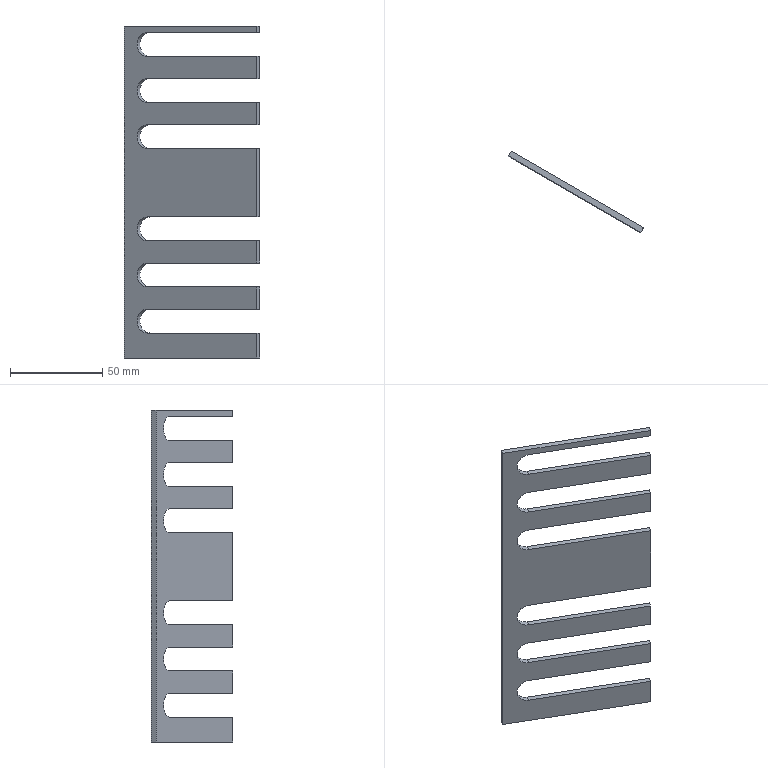Component | SolidWorks | KLHFH017AdjustmentShim-1 | 1 solid | 30 faces | box 73.38 x 44.1 x 180 mm | volume 27596 mm3 | plane 24 | cylinder 6 | commonest cylinder face diameters 13 x6 | material Plain Carbon Steel
STEP:
#1=COLOUR_RGB('',0.7922,0.8196,0.9333);
#2=FILL_AREA_STYLE_COLOUR('',#1);
#3=FILL_AREA_STYLE('',(#2));
#4=SURFACE_STYLE_FILL_AREA(#3);
#5=SURFACE_SIDE_STYLE('',(#4));
#6=SURFACE_STYLE_USAGE(.BOTH.,#5);
#7=PRESENTATION_STYLE_ASSIGNMENT((#6));
#8=CARTESIAN_POINT('',(6.04,7.196,-8.11));
#9=VERTEX_POINT('',#8);
#10=CARTESIAN_POINT('',(5.981,7.094,-8.11));
#11=VERTEX_POINT('',#10);
#12=CARTESIAN_POINT('',(6.04,7.196,-8.11));
#13=DIRECTION('',(-0.5,-0.866,0.));
#14=VECTOR('',#13,39.37);
#15=LINE('',#12,#14);
#16=EDGE_CURVE('',#9,#11,#15,.T.);
#17=ORIENTED_EDGE('',*,*,#16,.F.);
#18=CARTESIAN_POINT('',(6.04,7.196,-7.638));
#19=VERTEX_POINT('',#18);
#20=CARTESIAN_POINT('',(6.04,7.196,-14.075));
#21=DIRECTION('',(0.,0.,1.));
#22=VECTOR('',#21,39.37);
#23=LINE('',#20,#22);
#24=EDGE_CURVE('',#9,#19,#23,.T.);
#25=ORIENTED_EDGE('',*,*,#24,.T.);
#26=CARTESIAN_POINT('',(5.981,7.094,-7.638));
#27=VERTEX_POINT('',#26);
#28=CARTESIAN_POINT('',(6.04,7.196,-7.638));
#29=DIRECTION('',(-0.5,-0.866,0.));
#30=VECTOR('',#29,39.37);
#31=LINE('',#28,#30);
#32=EDGE_CURVE('',#19,#27,#31,.T.);
#33=ORIENTED_EDGE('',*,*,#32,.T.);
#34=CARTESIAN_POINT('',(5.981,7.094,-14.075));
#35=DIRECTION('',(0.,0.,1.));
#36=VECTOR('',#35,39.37);
#37=LINE('',#34,#36);
#38=EDGE_CURVE('',#11,#27,#37,.T.);
#39=ORIENTED_EDGE('',*,*,#38,.F.);
#40=EDGE_LOOP('',(#17,#25,#33,#39));
#41=FACE_OUTER_BOUND('',#40,.T.);
#42=CARTESIAN_POINT('',(5.981,7.094,-14.075));
#43=DIRECTION('',(0.866,-0.5,0.));
#44=DIRECTION('',(0.,0.,1.));
#45=AXIS2_PLACEMENT_3D('',#42,#43,#44);
#46=PLANE('',#45);
#47=ADVANCED_FACE('',(#41),#46,.T.);
#48=CARTESIAN_POINT('',(6.04,7.196,-13.031));
#49=VERTEX_POINT('',#48);
#50=CARTESIAN_POINT('',(3.704,8.545,-13.031));
#51=VERTEX_POINT('',#50);
#52=CARTESIAN_POINT('',(3.704,8.545,-13.031));
#53=DIRECTION('',(-0.866,0.5,0.));
#54=VECTOR('',#53,39.37);
#55=LINE('',#52,#54);
#56=EDGE_CURVE('',#49,#51,#55,.T.);
#57=ORIENTED_EDGE('',*,*,#56,.T.);
#58=CARTESIAN_POINT('',(3.704,8.545,-13.543));
#59=VERTEX_POINT('',#58);
#60=CARTESIAN_POINT('',(3.704,8.545,-13.287));
#61=DIRECTION('',(-0.5,-0.866,0.));
#62=DIRECTION('',(0.,0.,-1.));
#63=AXIS2_PLACEMENT_3D('',#60,#61,#62);
#64=CIRCLE('',#63,0.2559);
#65=EDGE_CURVE('',#51,#59,#64,.T.);
#66=ORIENTED_EDGE('',*,*,#65,.T.);
#67=CARTESIAN_POINT('',(6.04,7.196,-13.543));
#68=VERTEX_POINT('',#67);
#69=CARTESIAN_POINT('',(3.704,8.545,-13.543));
#70=DIRECTION('',(0.866,-0.5,0.));
#71=VECTOR('',#70,39.37);
#72=LINE('',#69,#71);
#73=EDGE_CURVE('',#59,#68,#72,.T.);
#74=ORIENTED_EDGE('',*,*,#73,.T.);
#75=CARTESIAN_POINT('',(6.04,7.196,-14.075));
#76=VERTEX_POINT('',#75);
#77=CARTESIAN_POINT('',(6.04,7.196,-14.075));
#78=DIRECTION('',(0.,0.,1.));
#79=VECTOR('',#78,39.37);
#80=LINE('',#77,#79);
#81=EDGE_CURVE('',#76,#68,#80,.T.);
#82=ORIENTED_EDGE('',*,*,#81,.F.);
#83=CARTESIAN_POINT('',(3.21,8.83,-14.075));
#84=VERTEX_POINT('',#83);
#85=CARTESIAN_POINT('',(3.21,8.83,-14.075));
#86=DIRECTION('',(-0.866,0.5,0.));
#87=VECTOR('',#86,39.37);
#88=LINE('',#85,#87);
#89=EDGE_CURVE('',#76,#84,#88,.T.);
#90=ORIENTED_EDGE('',*,*,#89,.T.);
#91=CARTESIAN_POINT('',(3.21,8.83,-6.988));
#92=VERTEX_POINT('',#91);
#93=CARTESIAN_POINT('',(3.21,8.83,-14.075));
#94=DIRECTION('',(0.,0.,1.));
#95=VECTOR('',#94,39.37);
#96=LINE('',#93,#95);
#97=EDGE_CURVE('',#84,#92,#96,.T.);
#98=ORIENTED_EDGE('',*,*,#97,.T.);
#99=CARTESIAN_POINT('',(6.04,7.196,-6.988));
#100=VERTEX_POINT('',#99);
#101=CARTESIAN_POINT('',(3.21,8.83,-6.988));
#102=DIRECTION('',(-0.866,0.5,0.));
#103=VECTOR('',#102,39.37);
#104=LINE('',#101,#103);
#105=EDGE_CURVE('',#100,#92,#104,.T.);
#106=ORIENTED_EDGE('',*,*,#105,.F.);
#107=CARTESIAN_POINT('',(6.04,7.196,-7.126));
#108=VERTEX_POINT('',#107);
#109=CARTESIAN_POINT('',(6.04,7.196,-14.075));
#110=DIRECTION('',(0.,0.,1.));
#111=VECTOR('',#110,39.37);
#112=LINE('',#109,#111);
#113=EDGE_CURVE('',#108,#100,#112,.T.);
#114=ORIENTED_EDGE('',*,*,#113,.F.);
#115=CARTESIAN_POINT('',(3.704,8.545,-7.126));
#116=VERTEX_POINT('',#115);
#117=CARTESIAN_POINT('',(3.704,8.545,-7.126));
#118=DIRECTION('',(-0.866,0.5,-0.));
#119=VECTOR('',#118,39.37);
#120=LINE('',#117,#119);
#121=EDGE_CURVE('',#108,#116,#120,.T.);
#122=ORIENTED_EDGE('',*,*,#121,.T.);
#123=CARTESIAN_POINT('',(3.704,8.545,-7.638));
#124=VERTEX_POINT('',#123);
#125=CARTESIAN_POINT('',(3.704,8.545,-7.382));
#126=DIRECTION('',(-0.5,-0.866,0.));
#127=DIRECTION('',(0.,0.,-1.));
#128=AXIS2_PLACEMENT_3D('',#125,#126,#127);
#129=CIRCLE('',#128,0.2559);
#130=EDGE_CURVE('',#116,#124,#129,.T.);
#131=ORIENTED_EDGE('',*,*,#130,.T.);
#132=CARTESIAN_POINT('',(3.704,8.545,-7.638));
#133=DIRECTION('',(0.866,-0.5,-0.));
#134=VECTOR('',#133,39.37);
#135=LINE('',#132,#134);
#136=EDGE_CURVE('',#124,#19,#135,.T.);
#137=ORIENTED_EDGE('',*,*,#136,.T.);
#138=ORIENTED_EDGE('',*,*,#24,.F.);
#139=CARTESIAN_POINT('',(3.704,8.545,-8.11));
#140=VERTEX_POINT('',#139);
#141=CARTESIAN_POINT('',(3.704,8.545,-8.11));
#142=DIRECTION('',(-0.866,0.5,0.));
#143=VECTOR('',#142,39.37);
#144=LINE('',#141,#143);
#145=EDGE_CURVE('',#9,#140,#144,.T.);
#146=ORIENTED_EDGE('',*,*,#145,.T.);
#147=CARTESIAN_POINT('',(3.704,8.545,-8.622));
#148=VERTEX_POINT('',#147);
#149=CARTESIAN_POINT('',(3.704,8.545,-8.366));
#150=DIRECTION('',(-0.5,-0.866,0.));
#151=DIRECTION('',(0.,0.,-1.));
#152=AXIS2_PLACEMENT_3D('',#149,#150,#151);
#153=CIRCLE('',#152,0.2559);
#154=EDGE_CURVE('',#140,#148,#153,.T.);
#155=ORIENTED_EDGE('',*,*,#154,.T.);
#156=CARTESIAN_POINT('',(6.04,7.196,-8.622));
#157=VERTEX_POINT('',#156);
#158=CARTESIAN_POINT('',(3.704,8.545,-8.622));
#159=DIRECTION('',(0.866,-0.5,0.));
#160=VECTOR('',#159,39.37);
#161=LINE('',#158,#160);
#162=EDGE_CURVE('',#148,#157,#161,.T.);
#163=ORIENTED_EDGE('',*,*,#162,.T.);
#164=CARTESIAN_POINT('',(6.04,7.196,-9.094));
#165=VERTEX_POINT('',#164);
#166=CARTESIAN_POINT('',(6.04,7.196,-14.075));
#167=DIRECTION('',(0.,0.,1.));
#168=VECTOR('',#167,39.37);
#169=LINE('',#166,#168);
#170=EDGE_CURVE('',#165,#157,#169,.T.);
#171=ORIENTED_EDGE('',*,*,#170,.F.);
#172=CARTESIAN_POINT('',(3.704,8.545,-9.094));
#173=VERTEX_POINT('',#172);
#174=CARTESIAN_POINT('',(3.704,8.545,-9.094));
#175=DIRECTION('',(-0.866,0.5,0.));
#176=VECTOR('',#175,39.37);
#177=LINE('',#174,#176);
#178=EDGE_CURVE('',#165,#173,#177,.T.);
#179=ORIENTED_EDGE('',*,*,#178,.T.);
#180=CARTESIAN_POINT('',(3.704,8.545,-9.606));
#181=VERTEX_POINT('',#180);
#182=CARTESIAN_POINT('',(3.704,8.545,-9.35));
#183=DIRECTION('',(-0.5,-0.866,0.));
#184=DIRECTION('',(0.,0.,-1.));
#185=AXIS2_PLACEMENT_3D('',#182,#183,#184);
#186=CIRCLE('',#185,0.2559);
#187=EDGE_CURVE('',#173,#181,#186,.T.);
#188=ORIENTED_EDGE('',*,*,#187,.T.);
#189=CARTESIAN_POINT('',(6.04,7.196,-9.606));
#190=VERTEX_POINT('',#189);
#191=CARTESIAN_POINT('',(3.704,8.545,-9.606));
#192=DIRECTION('',(0.866,-0.5,0.));
#193=VECTOR('',#192,39.37);
#194=LINE('',#191,#193);
#195=EDGE_CURVE('',#181,#190,#194,.T.);
#196=ORIENTED_EDGE('',*,*,#195,.T.);
#197=CARTESIAN_POINT('',(6.04,7.196,-11.063));
#198=VERTEX_POINT('',#197);
#199=CARTESIAN_POINT('',(6.04,7.196,-14.075));
#200=DIRECTION('',(0.,0.,1.));
#201=VECTOR('',#200,39.37);
#202=LINE('',#199,#201);
#203=EDGE_CURVE('',#198,#190,#202,.T.);
#204=ORIENTED_EDGE('',*,*,#203,.F.);
#205=CARTESIAN_POINT('',(3.704,8.545,-11.063));
#206=VERTEX_POINT('',#205);
#207=CARTESIAN_POINT('',(3.704,8.545,-11.063));
#208=DIRECTION('',(-0.866,0.5,0.));
#209=VECTOR('',#208,39.37);
#210=LINE('',#207,#209);
#211=EDGE_CURVE('',#198,#206,#210,.T.);
#212=ORIENTED_EDGE('',*,*,#211,.T.);
#213=CARTESIAN_POINT('',(3.704,8.545,-11.575));
#214=VERTEX_POINT('',#213);
#215=CARTESIAN_POINT('',(3.704,8.545,-11.319));
#216=DIRECTION('',(-0.5,-0.866,0.));
#217=DIRECTION('',(0.,0.,-1.));
#218=AXIS2_PLACEMENT_3D('',#215,#216,#217);
#219=CIRCLE('',#218,0.2559);
#220=EDGE_CURVE('',#206,#214,#219,.T.);
#221=ORIENTED_EDGE('',*,*,#220,.T.);
#222=CARTESIAN_POINT('',(6.04,7.196,-11.575));
#223=VERTEX_POINT('',#222);
#224=CARTESIAN_POINT('',(3.704,8.545,-11.575));
#225=DIRECTION('',(0.866,-0.5,0.));
#226=VECTOR('',#225,39.37);
#227=LINE('',#224,#226);
#228=EDGE_CURVE('',#214,#223,#227,.T.);
#229=ORIENTED_EDGE('',*,*,#228,.T.);
#230=CARTESIAN_POINT('',(6.04,7.196,-12.047));
#231=VERTEX_POINT('',#230);
#232=CARTESIAN_POINT('',(6.04,7.196,-14.075));
#233=DIRECTION('',(0.,0.,1.));
#234=VECTOR('',#233,39.37);
#235=LINE('',#232,#234);
#236=EDGE_CURVE('',#231,#223,#235,.T.);
#237=ORIENTED_EDGE('',*,*,#236,.F.);
#238=CARTESIAN_POINT('',(3.704,8.545,-12.047));
#239=VERTEX_POINT('',#238);
#240=CARTESIAN_POINT('',(3.704,8.545,-12.047));
#241=DIRECTION('',(-0.866,0.5,0.));
#242=VECTOR('',#241,39.37);
#243=LINE('',#240,#242);
#244=EDGE_CURVE('',#231,#239,#243,.T.);
#245=ORIENTED_EDGE('',*,*,#244,.T.);
#246=CARTESIAN_POINT('',(3.704,8.545,-12.559));
#247=VERTEX_POINT('',#246);
#248=CARTESIAN_POINT('',(3.704,8.545,-12.303));
#249=DIRECTION('',(-0.5,-0.866,0.));
#250=DIRECTION('',(0.,0.,-1.));
#251=AXIS2_PLACEMENT_3D('',#248,#249,#250);
#252=CIRCLE('',#251,0.2559);
#253=EDGE_CURVE('',#239,#247,#252,.T.);
#254=ORIENTED_EDGE('',*,*,#253,.T.);
#255=CARTESIAN_POINT('',(6.04,7.196,-12.559));
#256=VERTEX_POINT('',#255);
#257=CARTESIAN_POINT('',(3.704,8.545,-12.559));
#258=DIRECTION('',(0.866,-0.5,0.));
#259=VECTOR('',#258,39.37);
#260=LINE('',#257,#259);
#261=EDGE_CURVE('',#247,#256,#260,.T.);
#262=ORIENTED_EDGE('',*,*,#261,.T.);
#263=CARTESIAN_POINT('',(6.04,7.196,-14.075));
#264=DIRECTION('',(0.,0.,1.));
#265=VECTOR('',#264,39.37);
#266=LINE('',#263,#265);
#267=EDGE_CURVE('',#49,#256,#266,.T.);
#268=ORIENTED_EDGE('',*,*,#267,.F.);
#269=EDGE_LOOP('',(#57,#66,#74,#82,#90,#98,#106,#114,#122,#131,#137,#138,#146,#155,#163,#171,#179,#188,#196,#204,#212,#221,#229,#237,#245,#254,#262,#268));
#270=FACE_OUTER_BOUND('',#269,.T.);
#271=CARTESIAN_POINT('',(3.21,8.83,-14.075));
#272=DIRECTION('',(0.5,0.866,-0.));
#273=DIRECTION('',(0.,0.,1.));
#274=AXIS2_PLACEMENT_3D('',#271,#272,#273);
#275=PLANE('',#274);
#276=ADVANCED_FACE('',(#270),#275,.T.);
#277=CARTESIAN_POINT('',(5.981,7.094,-12.047));
#278=VERTEX_POINT('',#277);
#279=CARTESIAN_POINT('',(6.04,7.196,-12.047));
#280=DIRECTION('',(-0.5,-0.866,0.));
#281=VECTOR('',#280,39.37);
#282=LINE('',#279,#281);
#283=EDGE_CURVE('',#231,#278,#282,.T.);
#284=ORIENTED_EDGE('',*,*,#283,.F.);
#285=ORIENTED_EDGE('',*,*,#236,.T.);
#286=CARTESIAN_POINT('',(5.981,7.094,-11.575));
#287=VERTEX_POINT('',#286);
#288=CARTESIAN_POINT('',(6.04,7.196,-11.575));
#289=DIRECTION('',(-0.5,-0.866,0.));
#290=VECTOR('',#289,39.37);
#291=LINE('',#288,#290);
#292=EDGE_CURVE('',#223,#287,#291,.T.);
#293=ORIENTED_EDGE('',*,*,#292,.T.);
#294=CARTESIAN_POINT('',(5.981,7.094,-14.075));
#295=DIRECTION('',(0.,0.,1.));
#296=VECTOR('',#295,39.37);
#297=LINE('',#294,#296);
#298=EDGE_CURVE('',#278,#287,#297,.T.);
#299=ORIENTED_EDGE('',*,*,#298,.F.);
#300=EDGE_LOOP('',(#284,#285,#293,#299));
#301=FACE_OUTER_BOUND('',#300,.T.);
#302=CARTESIAN_POINT('',(5.981,7.094,-14.075));
#303=DIRECTION('',(0.866,-0.5,0.));
#304=DIRECTION('',(0.,0.,1.));
#305=AXIS2_PLACEMENT_3D('',#302,#303,#304);
#306=PLANE('',#305);
#307=ADVANCED_FACE('',(#301),#306,.T.);
#308=CARTESIAN_POINT('',(3.645,8.442,-13.031));
#309=VERTEX_POINT('',#308);
#310=CARTESIAN_POINT('',(3.645,8.442,-13.543));
#311=VERTEX_POINT('',#310);
#312=CARTESIAN_POINT('',(3.645,8.442,-13.287));
#313=DIRECTION('',(-0.5,-0.866,0.));
#314=DIRECTION('',(0.,0.,-1.));
#315=AXIS2_PLACEMENT_3D('',#312,#313,#314);
#316=CIRCLE('',#315,0.2559);
#317=EDGE_CURVE('',#309,#311,#316,.T.);
#318=ORIENTED_EDGE('',*,*,#317,.F.);
#319=CARTESIAN_POINT('',(5.981,7.094,-13.031));
#320=VERTEX_POINT('',#319);
#321=CARTESIAN_POINT('',(3.645,8.442,-13.031));
#322=DIRECTION('',(-0.866,0.5,0.));
#323=VECTOR('',#322,39.37);
#324=LINE('',#321,#323);
#325=EDGE_CURVE('',#320,#309,#324,.T.);
#326=ORIENTED_EDGE('',*,*,#325,.F.);
#327=CARTESIAN_POINT('',(5.981,7.094,-12.559));
#328=VERTEX_POINT('',#327);
#329=CARTESIAN_POINT('',(5.981,7.094,-14.075));
#330=DIRECTION('',(0.,0.,1.));
#331=VECTOR('',#330,39.37);
#332=LINE('',#329,#331);
#333=EDGE_CURVE('',#320,#328,#332,.T.);
#334=ORIENTED_EDGE('',*,*,#333,.T.);
#335=CARTESIAN_POINT('',(3.645,8.442,-12.559));
#336=VERTEX_POINT('',#335);
#337=CARTESIAN_POINT('',(3.645,8.442,-12.559));
#338=DIRECTION('',(0.866,-0.5,0.));
#339=VECTOR('',#338,39.37);
#340=LINE('',#337,#339);
#341=EDGE_CURVE('',#336,#328,#340,.T.);
#342=ORIENTED_EDGE('',*,*,#341,.F.);
#343=CARTESIAN_POINT('',(3.645,8.442,-12.047));
#344=VERTEX_POINT('',#343);
#345=CARTESIAN_POINT('',(3.645,8.442,-12.303));
#346=DIRECTION('',(-0.5,-0.866,0.));
#347=DIRECTION('',(0.,0.,-1.));
#348=AXIS2_PLACEMENT_3D('',#345,#346,#347);
#349=CIRCLE('',#348,0.2559);
#350=EDGE_CURVE('',#344,#336,#349,.T.);
#351=ORIENTED_EDGE('',*,*,#350,.F.);
#352=CARTESIAN_POINT('',(3.645,8.442,-12.047));
#353=DIRECTION('',(-0.866,0.5,0.));
#354=VECTOR('',#353,39.37);
#355=LINE('',#352,#354);
#356=EDGE_CURVE('',#278,#344,#355,.T.);
#357=ORIENTED_EDGE('',*,*,#356,.F.);
#358=ORIENTED_EDGE('',*,*,#298,.T.);
#359=CARTESIAN_POINT('',(3.645,8.442,-11.575));
#360=VERTEX_POINT('',#359);
#361=CARTESIAN_POINT('',(3.645,8.442,-11.575));
#362=DIRECTION('',(0.866,-0.5,0.));
#363=VECTOR('',#362,39.37);
#364=LINE('',#361,#363);
#365=EDGE_CURVE('',#360,#287,#364,.T.);
#366=ORIENTED_EDGE('',*,*,#365,.F.);
#367=CARTESIAN_POINT('',(3.645,8.442,-11.063));
#368=VERTEX_POINT('',#367);
#369=CARTESIAN_POINT('',(3.645,8.442,-11.319));
#370=DIRECTION('',(-0.5,-0.866,0.));
#371=DIRECTION('',(0.,0.,-1.));
#372=AXIS2_PLACEMENT_3D('',#369,#370,#371);
#373=CIRCLE('',#372,0.2559);
#374=EDGE_CURVE('',#368,#360,#373,.T.);
#375=ORIENTED_EDGE('',*,*,#374,.F.);
#376=CARTESIAN_POINT('',(5.981,7.094,-11.063));
#377=VERTEX_POINT('',#376);
#378=CARTESIAN_POINT('',(3.645,8.442,-11.063));
#379=DIRECTION('',(-0.866,0.5,0.));
#380=VECTOR('',#379,39.37);
#381=LINE('',#378,#380);
#382=EDGE_CURVE('',#377,#368,#381,.T.);
#383=ORIENTED_EDGE('',*,*,#382,.F.);
#384=CARTESIAN_POINT('',(5.981,7.094,-9.606));
#385=VERTEX_POINT('',#384);
#386=CARTESIAN_POINT('',(5.981,7.094,-14.075));
#387=DIRECTION('',(0.,0.,1.));
#388=VECTOR('',#387,39.37);
#389=LINE('',#386,#388);
#390=EDGE_CURVE('',#377,#385,#389,.T.);
#391=ORIENTED_EDGE('',*,*,#390,.T.);
#392=CARTESIAN_POINT('',(3.645,8.442,-9.606));
#393=VERTEX_POINT('',#392);
#394=CARTESIAN_POINT('',(3.645,8.442,-9.606));
#395=DIRECTION('',(0.866,-0.5,0.));
#396=VECTOR('',#395,39.37);
#397=LINE('',#394,#396);
#398=EDGE_CURVE('',#393,#385,#397,.T.);
#399=ORIENTED_EDGE('',*,*,#398,.F.);
#400=CARTESIAN_POINT('',(3.645,8.442,-9.094));
#401=VERTEX_POINT('',#400);
#402=CARTESIAN_POINT('',(3.645,8.442,-9.35));
#403=DIRECTION('',(-0.5,-0.866,0.));
#404=DIRECTION('',(0.,0.,-1.));
#405=AXIS2_PLACEMENT_3D('',#402,#403,#404);
#406=CIRCLE('',#405,0.2559);
#407=EDGE_CURVE('',#401,#393,#406,.T.);
#408=ORIENTED_EDGE('',*,*,#407,.F.);
#409=CARTESIAN_POINT('',(5.981,7.094,-9.094));
#410=VERTEX_POINT('',#409);
#411=CARTESIAN_POINT('',(3.645,8.442,-9.094));
#412=DIRECTION('',(-0.866,0.5,0.));
#413=VECTOR('',#412,39.37);
#414=LINE('',#411,#413);
#415=EDGE_CURVE('',#410,#401,#414,.T.);
#416=ORIENTED_EDGE('',*,*,#415,.F.);
#417=CARTESIAN_POINT('',(5.981,7.094,-8.622));
#418=VERTEX_POINT('',#417);
#419=CARTESIAN_POINT('',(5.981,7.094,-14.075));
#420=DIRECTION('',(0.,0.,1.));
#421=VECTOR('',#420,39.37);
#422=LINE('',#419,#421);
#423=EDGE_CURVE('',#410,#418,#422,.T.);
#424=ORIENTED_EDGE('',*,*,#423,.T.);
#425=CARTESIAN_POINT('',(3.645,8.442,-8.622));
#426=VERTEX_POINT('',#425);
#427=CARTESIAN_POINT('',(3.645,8.442,-8.622));
#428=DIRECTION('',(0.866,-0.5,0.));
#429=VECTOR('',#428,39.37);
#430=LINE('',#427,#429);
#431=EDGE_CURVE('',#426,#418,#430,.T.);
#432=ORIENTED_EDGE('',*,*,#431,.F.);
#433=CARTESIAN_POINT('',(3.645,8.442,-8.11));
#434=VERTEX_POINT('',#433);
#435=CARTESIAN_POINT('',(3.645,8.442,-8.366));
#436=DIRECTION('',(-0.5,-0.866,0.));
#437=DIRECTION('',(0.,0.,-1.));
#438=AXIS2_PLACEMENT_3D('',#435,#436,#437);
#439=CIRCLE('',#438,0.2559);
#440=EDGE_CURVE('',#434,#426,#439,.T.);
#441=ORIENTED_EDGE('',*,*,#440,.F.);
#442=CARTESIAN_POINT('',(3.645,8.442,-8.11));
#443=DIRECTION('',(-0.866,0.5,0.));
#444=VECTOR('',#443,39.37);
#445=LINE('',#442,#444);
#446=EDGE_CURVE('',#11,#434,#445,.T.);
#447=ORIENTED_EDGE('',*,*,#446,.F.);
#448=ORIENTED_EDGE('',*,*,#38,.T.);
#449=CARTESIAN_POINT('',(3.645,8.442,-7.638));
#450=VERTEX_POINT('',#449);
#451=CARTESIAN_POINT('',(3.645,8.442,-7.638));
#452=DIRECTION('',(0.866,-0.5,-0.));
#453=VECTOR('',#452,39.37);
#454=LINE('',#451,#453);
#455=EDGE_CURVE('',#450,#27,#454,.T.);
#456=ORIENTED_EDGE('',*,*,#455,.F.);
#457=CARTESIAN_POINT('',(3.645,8.442,-7.126));
#458=VERTEX_POINT('',#457);
#459=CARTESIAN_POINT('',(3.645,8.442,-7.382));
#460=DIRECTION('',(-0.5,-0.866,0.));
#461=DIRECTION('',(0.,0.,-1.));
#462=AXIS2_PLACEMENT_3D('',#459,#460,#461);
#463=CIRCLE('',#462,0.2559);
#464=EDGE_CURVE('',#458,#450,#463,.T.);
#465=ORIENTED_EDGE('',*,*,#464,.F.);
#466=CARTESIAN_POINT('',(5.981,7.094,-7.126));
#467=VERTEX_POINT('',#466);
#468=CARTESIAN_POINT('',(3.645,8.442,-7.126));
#469=DIRECTION('',(-0.866,0.5,-0.));
#470=VECTOR('',#469,39.37);
#471=LINE('',#468,#470);
#472=EDGE_CURVE('',#467,#458,#471,.T.);
#473=ORIENTED_EDGE('',*,*,#472,.F.);
#474=CARTESIAN_POINT('',(5.981,7.094,-6.988));
#475=VERTEX_POINT('',#474);
#476=CARTESIAN_POINT('',(5.981,7.094,-14.075));
#477=DIRECTION('',(0.,0.,1.));
#478=VECTOR('',#477,39.37);
#479=LINE('',#476,#478);
#480=EDGE_CURVE('',#467,#475,#479,.T.);
#481=ORIENTED_EDGE('',*,*,#480,.T.);
#482=CARTESIAN_POINT('',(3.151,8.728,-6.988));
#483=VERTEX_POINT('',#482);
#484=CARTESIAN_POINT('',(3.151,8.728,-6.988));
#485=DIRECTION('',(-0.866,0.5,0.));
#486=VECTOR('',#485,39.37);
#487=LINE('',#484,#486);
#488=EDGE_CURVE('',#475,#483,#487,.T.);
#489=ORIENTED_EDGE('',*,*,#488,.T.);
#490=CARTESIAN_POINT('',(3.151,8.728,-14.075));
#491=VERTEX_POINT('',#490);
#492=CARTESIAN_POINT('',(3.151,8.728,-14.075));
#493=DIRECTION('',(0.,0.,1.));
#494=VECTOR('',#493,39.37);
#495=LINE('',#492,#494);
#496=EDGE_CURVE('',#491,#483,#495,.T.);
#497=ORIENTED_EDGE('',*,*,#496,.F.);
#498=CARTESIAN_POINT('',(5.981,7.094,-14.075));
#499=VERTEX_POINT('',#498);
#500=CARTESIAN_POINT('',(3.151,8.728,-14.075));
#501=DIRECTION('',(-0.866,0.5,0.));
#502=VECTOR('',#501,39.37);
#503=LINE('',#500,#502);
#504=EDGE_CURVE('',#499,#491,#503,.T.);
#505=ORIENTED_EDGE('',*,*,#504,.F.);
#506=CARTESIAN_POINT('',(5.981,7.094,-13.543));
#507=VERTEX_POINT('',#506);
#508=CARTESIAN_POINT('',(5.981,7.094,-14.075));
#509=DIRECTION('',(0.,0.,1.));
#510=VECTOR('',#509,39.37);
#511=LINE('',#508,#510);
#512=EDGE_CURVE('',#499,#507,#511,.T.);
#513=ORIENTED_EDGE('',*,*,#512,.T.);
#514=CARTESIAN_POINT('',(3.645,8.442,-13.543));
#515=DIRECTION('',(0.866,-0.5,0.));
#516=VECTOR('',#515,39.37);
#517=LINE('',#514,#516);
#518=EDGE_CURVE('',#311,#507,#517,.T.);
#519=ORIENTED_EDGE('',*,*,#518,.F.);
#520=EDGE_LOOP('',(#318,#326,#334,#342,#351,#357,#358,#366,#375,#383,#391,#399,#408,#416,#424,#432,#441,#447,#448,#456,#465,#473,#481,#489,#497,#505,#513,#519));
#521=FACE_OUTER_BOUND('',#520,.T.);
#522=CARTESIAN_POINT('',(3.151,8.728,-14.075));
#523=DIRECTION('',(0.5,0.866,-0.));
#524=DIRECTION('',(0.,0.,1.));
#525=AXIS2_PLACEMENT_3D('',#522,#523,#524);
#526=PLANE('',#525);
#527=ADVANCED_FACE('',(#521),#526,.F.);
#528=CARTESIAN_POINT('',(6.04,7.196,-7.126));
#529=DIRECTION('',(-0.5,-0.866,0.));
#530=VECTOR('',#529,39.37);
#531=LINE('',#528,#530);
#532=EDGE_CURVE('',#108,#467,#531,.T.);
#533=ORIENTED_EDGE('',*,*,#532,.F.);
#534=ORIENTED_EDGE('',*,*,#113,.T.);
#535=CARTESIAN_POINT('',(5.981,7.094,-6.988));
#536=DIRECTION('',(0.5,0.866,-0.));
#537=VECTOR('',#536,39.37);
#538=LINE('',#535,#537);
#539=EDGE_CURVE('',#475,#100,#538,.T.);
#540=ORIENTED_EDGE('',*,*,#539,.F.);
#541=ORIENTED_EDGE('',*,*,#480,.F.);
#542=EDGE_LOOP('',(#533,#534,#540,#541));
#543=FACE_OUTER_BOUND('',#542,.T.);
#544=CARTESIAN_POINT('',(5.981,7.094,-14.075));
#545=DIRECTION('',(0.866,-0.5,0.));
#546=DIRECTION('',(0.,0.,1.));
#547=AXIS2_PLACEMENT_3D('',#544,#545,#546);
#548=PLANE('',#547);
#549=ADVANCED_FACE('',(#543),#548,.T.);
#550=CARTESIAN_POINT('',(6.04,7.196,-9.094));
#551=DIRECTION('',(-0.5,-0.866,0.));
#552=VECTOR('',#551,39.37);
#553=LINE('',#550,#552);
#554=EDGE_CURVE('',#165,#410,#553,.T.);
#555=ORIENTED_EDGE('',*,*,#554,.F.);
#556=ORIENTED_EDGE('',*,*,#170,.T.);
#557=CARTESIAN_POINT('',(6.04,7.196,-8.622));
#558=DIRECTION('',(-0.5,-0.866,0.));
#559=VECTOR('',#558,39.37);
#560=LINE('',#557,#559);
#561=EDGE_CURVE('',#157,#418,#560,.T.);
#562=ORIENTED_EDGE('',*,*,#561,.T.);
#563=ORIENTED_EDGE('',*,*,#423,.F.);
#564=EDGE_LOOP('',(#555,#556,#562,#563));
#565=FACE_OUTER_BOUND('',#564,.T.);
#566=CARTESIAN_POINT('',(5.981,7.094,-14.075));
#567=DIRECTION('',(0.866,-0.5,0.));
#568=DIRECTION('',(0.,0.,1.));
#569=AXIS2_PLACEMENT_3D('',#566,#567,#568);
#570=PLANE('',#569);
#571=ADVANCED_FACE('',(#565),#570,.T.);
#572=CARTESIAN_POINT('',(6.04,7.196,-11.063));
#573=DIRECTION('',(-0.5,-0.866,0.));
#574=VECTOR('',#573,39.37);
#575=LINE('',#572,#574);
#576=EDGE_CURVE('',#198,#377,#575,.T.);
#577=ORIENTED_EDGE('',*,*,#576,.F.);
#578=ORIENTED_EDGE('',*,*,#203,.T.);
#579=CARTESIAN_POINT('',(6.04,7.196,-9.606));
#580=DIRECTION('',(-0.5,-0.866,0.));
#581=VECTOR('',#580,39.37);
#582=LINE('',#579,#581);
#583=EDGE_CURVE('',#190,#385,#582,.T.);
#584=ORIENTED_EDGE('',*,*,#583,.T.);
#585=ORIENTED_EDGE('',*,*,#390,.F.);
#586=EDGE_LOOP('',(#577,#578,#584,#585));
#587=FACE_OUTER_BOUND('',#586,.T.);
#588=CARTESIAN_POINT('',(5.981,7.094,-14.075));
#589=DIRECTION('',(0.866,-0.5,0.));
#590=DIRECTION('',(0.,0.,1.));
#591=AXIS2_PLACEMENT_3D('',#588,#589,#590);
#592=PLANE('',#591);
#593=ADVANCED_FACE('',(#587),#592,.T.);
#594=CARTESIAN_POINT('',(6.04,7.196,-13.031));
#595=DIRECTION('',(-0.5,-0.866,0.));
#596=VECTOR('',#595,39.37);
#597=LINE('',#594,#596);
#598=EDGE_CURVE('',#49,#320,#597,.T.);
#599=ORIENTED_EDGE('',*,*,#598,.F.);
#600=ORIENTED_EDGE('',*,*,#267,.T.);
#601=CARTESIAN_POINT('',(6.04,7.196,-12.559));
#602=DIRECTION('',(-0.5,-0.866,0.));
#603=VECTOR('',#602,39.37);
#604=LINE('',#601,#603);
#605=EDGE_CURVE('',#256,#328,#604,.T.);
#606=ORIENTED_EDGE('',*,*,#605,.T.);
#607=ORIENTED_EDGE('',*,*,#333,.F.);
#608=EDGE_LOOP('',(#599,#600,#606,#607));
#609=FACE_OUTER_BOUND('',#608,.T.);
#610=CARTESIAN_POINT('',(5.981,7.094,-14.075));
#611=DIRECTION('',(0.866,-0.5,0.));
#612=DIRECTION('',(0.,0.,1.));
#613=AXIS2_PLACEMENT_3D('',#610,#611,#612);
#614=PLANE('',#613);
#615=ADVANCED_FACE('',(#609),#614,.T.);
#616=CARTESIAN_POINT('',(3.21,8.83,-6.988));
#617=DIRECTION('',(-0.5,-0.866,0.));
#618=VECTOR('',#617,39.37);
#619=LINE('',#616,#618);
#620=EDGE_CURVE('',#92,#483,#619,.T.);
#621=ORIENTED_EDGE('',*,*,#620,.F.);
#622=ORIENTED_EDGE('',*,*,#97,.F.);
#623=CARTESIAN_POINT('',(3.21,8.83,-14.075));
#624=DIRECTION('',(-0.5,-0.866,0.));
#625=VECTOR('',#624,39.37);
#626=LINE('',#623,#625);
#627=EDGE_CURVE('',#84,#491,#626,.T.);
#628=ORIENTED_EDGE('',*,*,#627,.T.);
#629=ORIENTED_EDGE('',*,*,#496,.T.);
#630=EDGE_LOOP('',(#621,#622,#628,#629));
#631=FACE_OUTER_BOUND('',#630,.T.);
#632=CARTESIAN_POINT('',(3.21,8.83,-14.075));
#633=DIRECTION('',(-0.866,0.5,0.));
#634=DIRECTION('',(-0.,-0.,-1.));
#635=AXIS2_PLACEMENT_3D('',#632,#633,#634);
#636=PLANE('',#635);
#637=ADVANCED_FACE('',(#631),#636,.T.);
#638=CARTESIAN_POINT('',(6.04,7.196,-13.543));
#639=DIRECTION('',(-0.5,-0.866,0.));
#640=VECTOR('',#639,39.37);
#641=LINE('',#638,#640);
#642=EDGE_CURVE('',#68,#507,#641,.T.);
#643=ORIENTED_EDGE('',*,*,#642,.T.);
#644=ORIENTED_EDGE('',*,*,#512,.F.);
#645=CARTESIAN_POINT('',(5.981,7.094,-14.075));
#646=DIRECTION('',(0.5,0.866,-0.));
#647=VECTOR('',#646,39.37);
#648=LINE('',#645,#647);
#649=EDGE_CURVE('',#499,#76,#648,.T.);
#650=ORIENTED_EDGE('',*,*,#649,.T.);
#651=ORIENTED_EDGE('',*,*,#81,.T.);
#652=EDGE_LOOP('',(#643,#644,#650,#651));
#653=FACE_OUTER_BOUND('',#652,.T.);
#654=CARTESIAN_POINT('',(5.981,7.094,-14.075));
#655=DIRECTION('',(0.866,-0.5,0.));
#656=DIRECTION('',(0.,0.,1.));
#657=AXIS2_PLACEMENT_3D('',#654,#655,#656);
#658=PLANE('',#657);
#659=ADVANCED_FACE('',(#653),#658,.T.);
#660=ORIENTED_EDGE('',*,*,#504,.T.);
#661=ORIENTED_EDGE('',*,*,#627,.F.);
#662=ORIENTED_EDGE('',*,*,#89,.F.);
#663=ORIENTED_EDGE('',*,*,#649,.F.);
#664=EDGE_LOOP('',(#660,#661,#662,#663));
#665=FACE_OUTER_BOUND('',#664,.T.);
#666=CARTESIAN_POINT('',(3.21,8.83,-14.075));
#667=DIRECTION('',(-0.,-0.,-1.));
#668=DIRECTION('',(0.866,-0.5,0.));
#669=AXIS2_PLACEMENT_3D('',#666,#667,#668);
#670=PLANE('',#669);
#671=ADVANCED_FACE('',(#665),#670,.T.);
#672=ORIENTED_EDGE('',*,*,#488,.F.);
#673=ORIENTED_EDGE('',*,*,#539,.T.);
#674=ORIENTED_EDGE('',*,*,#105,.T.);
#675=ORIENTED_EDGE('',*,*,#620,.T.);
#676=EDGE_LOOP('',(#672,#673,#674,#675));
#677=FACE_OUTER_BOUND('',#676,.T.);
#678=CARTESIAN_POINT('',(3.21,8.83,-6.988));
#679=DIRECTION('',(-0.,-0.,-1.));
#680=DIRECTION('',(0.866,-0.5,0.));
#681=AXIS2_PLACEMENT_3D('',#678,#679,#680);
#682=PLANE('',#681);
#683=ADVANCED_FACE('',(#677),#682,.F.);
#684=ORIENTED_EDGE('',*,*,#464,.T.);
#685=CARTESIAN_POINT('',(3.704,8.545,-7.638));
#686=DIRECTION('',(-0.5,-0.866,0.));
#687=VECTOR('',#686,39.37);
#688=LINE('',#685,#687);
#689=EDGE_CURVE('',#124,#450,#688,.T.);
#690=ORIENTED_EDGE('',*,*,#689,.F.);
#691=ORIENTED_EDGE('',*,*,#130,.F.);
#692=CARTESIAN_POINT('',(3.704,8.545,-7.126));
#693=DIRECTION('',(-0.5,-0.866,0.));
#694=VECTOR('',#693,39.37);
#695=LINE('',#692,#694);
#696=EDGE_CURVE('',#116,#458,#695,.T.);
#697=ORIENTED_EDGE('',*,*,#696,.T.);
#698=EDGE_LOOP('',(#684,#690,#691,#697));
#699=FACE_OUTER_BOUND('',#698,.T.);
#700=CARTESIAN_POINT('',(3.704,8.545,-7.382));
#701=DIRECTION('',(-0.5,-0.866,0.));
#702=DIRECTION('',(0.,0.,-1.));
#703=AXIS2_PLACEMENT_3D('',#700,#701,#702);
#704=CYLINDRICAL_SURFACE('',#703,0.2559);
#705=ADVANCED_FACE('',(#699),#704,.F.);
#706=ORIENTED_EDGE('',*,*,#472,.T.);
#707=ORIENTED_EDGE('',*,*,#696,.F.);
#708=ORIENTED_EDGE('',*,*,#121,.F.);
#709=ORIENTED_EDGE('',*,*,#532,.T.);
#710=EDGE_LOOP('',(#706,#707,#708,#709));
#711=FACE_OUTER_BOUND('',#710,.T.);
#712=CARTESIAN_POINT('',(3.704,8.545,-7.126));
#713=DIRECTION('',(-0.,0.,1.));
#714=DIRECTION('',(-0.866,0.5,-0.));
#715=AXIS2_PLACEMENT_3D('',#712,#713,#714);
#716=PLANE('',#715);
#717=ADVANCED_FACE('',(#711),#716,.F.);
#718=ORIENTED_EDGE('',*,*,#455,.T.);
#719=ORIENTED_EDGE('',*,*,#32,.F.);
#720=ORIENTED_EDGE('',*,*,#136,.F.);
#721=ORIENTED_EDGE('',*,*,#689,.T.);
#722=EDGE_LOOP('',(#718,#719,#720,#721));
#723=FACE_OUTER_BOUND('',#722,.T.);
#724=CARTESIAN_POINT('',(3.704,8.545,-7.638));
#725=DIRECTION('',(-0.,0.,-1.));
#726=DIRECTION('',(0.866,-0.5,-0.));
#727=AXIS2_PLACEMENT_3D('',#724,#725,#726);
#728=PLANE('',#727);
#729=ADVANCED_FACE('',(#723),#728,.F.);
#730=ORIENTED_EDGE('',*,*,#440,.T.);
#731=CARTESIAN_POINT('',(3.704,8.545,-8.622));
#732=DIRECTION('',(-0.5,-0.866,0.));
#733=VECTOR('',#732,39.37);
#734=LINE('',#731,#733);
#735=EDGE_CURVE('',#148,#426,#734,.T.);
#736=ORIENTED_EDGE('',*,*,#735,.F.);
#737=ORIENTED_EDGE('',*,*,#154,.F.);
#738=CARTESIAN_POINT('',(3.704,8.545,-8.11));
#739=DIRECTION('',(-0.5,-0.866,0.));
#740=VECTOR('',#739,39.37);
#741=LINE('',#738,#740);
#742=EDGE_CURVE('',#140,#434,#741,.T.);
#743=ORIENTED_EDGE('',*,*,#742,.T.);
#744=EDGE_LOOP('',(#730,#736,#737,#743));
#745=FACE_OUTER_BOUND('',#744,.T.);
#746=CARTESIAN_POINT('',(3.704,8.545,-8.366));
#747=DIRECTION('',(-0.5,-0.866,0.));
#748=DIRECTION('',(0.,0.,-1.));
#749=AXIS2_PLACEMENT_3D('',#746,#747,#748);
#750=CYLINDRICAL_SURFACE('',#749,0.2559);
#751=ADVANCED_FACE('',(#745),#750,.F.);
#752=ORIENTED_EDGE('',*,*,#446,.T.);
#753=ORIENTED_EDGE('',*,*,#742,.F.);
#754=ORIENTED_EDGE('',*,*,#145,.F.);
#755=ORIENTED_EDGE('',*,*,#16,.T.);
#756=EDGE_LOOP('',(#752,#753,#754,#755));
#757=FACE_OUTER_BOUND('',#756,.T.);
#758=CARTESIAN_POINT('',(3.704,8.545,-8.11));
#759=DIRECTION('',(0.,0.,1.));
#760=DIRECTION('',(-0.866,0.5,0.));
#761=AXIS2_PLACEMENT_3D('',#758,#759,#760);
#762=PLANE('',#761);
#763=ADVANCED_FACE('',(#757),#762,.F.);
#764=ORIENTED_EDGE('',*,*,#431,.T.);
#765=ORIENTED_EDGE('',*,*,#561,.F.);
#766=ORIENTED_EDGE('',*,*,#162,.F.);
#767=ORIENTED_EDGE('',*,*,#735,.T.);
#768=EDGE_LOOP('',(#764,#765,#766,#767));
#769=FACE_OUTER_BOUND('',#768,.T.);
#770=CARTESIAN_POINT('',(3.704,8.545,-8.622));
#771=DIRECTION('',(-0.,-0.,-1.));
#772=DIRECTION('',(0.866,-0.5,0.));
#773=AXIS2_PLACEMENT_3D('',#770,#771,#772);
#774=PLANE('',#773);
#775=ADVANCED_FACE('',(#769),#774,.F.);
#776=ORIENTED_EDGE('',*,*,#407,.T.);
#777=CARTESIAN_POINT('',(3.704,8.545,-9.606));
#778=DIRECTION('',(-0.5,-0.866,0.));
#779=VECTOR('',#778,39.37);
#780=LINE('',#777,#779);
#781=EDGE_CURVE('',#181,#393,#780,.T.);
#782=ORIENTED_EDGE('',*,*,#781,.F.);
#783=ORIENTED_EDGE('',*,*,#187,.F.);
#784=CARTESIAN_POINT('',(3.704,8.545,-9.094));
#785=DIRECTION('',(-0.5,-0.866,0.));
#786=VECTOR('',#785,39.37);
#787=LINE('',#784,#786);
#788=EDGE_CURVE('',#173,#401,#787,.T.);
#789=ORIENTED_EDGE('',*,*,#788,.T.);
#790=EDGE_LOOP('',(#776,#782,#783,#789));
#791=FACE_OUTER_BOUND('',#790,.T.);
#792=CARTESIAN_POINT('',(3.704,8.545,-9.35));
#793=DIRECTION('',(-0.5,-0.866,0.));
#794=DIRECTION('',(0.,0.,-1.));
#795=AXIS2_PLACEMENT_3D('',#792,#793,#794);
#796=CYLINDRICAL_SURFACE('',#795,0.2559);
#797=ADVANCED_FACE('',(#791),#796,.F.);
#798=ORIENTED_EDGE('',*,*,#415,.T.);
#799=ORIENTED_EDGE('',*,*,#788,.F.);
#800=ORIENTED_EDGE('',*,*,#178,.F.);
#801=ORIENTED_EDGE('',*,*,#554,.T.);
#802=EDGE_LOOP('',(#798,#799,#800,#801));
#803=FACE_OUTER_BOUND('',#802,.T.);
#804=CARTESIAN_POINT('',(3.704,8.545,-9.094));
#805=DIRECTION('',(0.,0.,1.));
#806=DIRECTION('',(-0.866,0.5,0.));
#807=AXIS2_PLACEMENT_3D('',#804,#805,#806);
#808=PLANE('',#807);
#809=ADVANCED_FACE('',(#803),#808,.F.);
#810=ORIENTED_EDGE('',*,*,#398,.T.);
#811=ORIENTED_EDGE('',*,*,#583,.F.);
#812=ORIENTED_EDGE('',*,*,#195,.F.);
#813=ORIENTED_EDGE('',*,*,#781,.T.);
#814=EDGE_LOOP('',(#810,#811,#812,#813));
#815=FACE_OUTER_BOUND('',#814,.T.);
#816=CARTESIAN_POINT('',(3.704,8.545,-9.606));
#817=DIRECTION('',(-0.,-0.,-1.));
#818=DIRECTION('',(0.866,-0.5,0.));
#819=AXIS2_PLACEMENT_3D('',#816,#817,#818);
#820=PLANE('',#819);
#821=ADVANCED_FACE('',(#815),#820,.F.);
#822=ORIENTED_EDGE('',*,*,#374,.T.);
#823=CARTESIAN_POINT('',(3.704,8.545,-11.575));
#824=DIRECTION('',(-0.5,-0.866,0.));
#825=VECTOR('',#824,39.37);
#826=LINE('',#823,#825);
#827=EDGE_CURVE('',#214,#360,#826,.T.);
#828=ORIENTED_EDGE('',*,*,#827,.F.);
#829=ORIENTED_EDGE('',*,*,#220,.F.);
#830=CARTESIAN_POINT('',(3.704,8.545,-11.063));
#831=DIRECTION('',(-0.5,-0.866,0.));
#832=VECTOR('',#831,39.37);
#833=LINE('',#830,#832);
#834=EDGE_CURVE('',#206,#368,#833,.T.);
#835=ORIENTED_EDGE('',*,*,#834,.T.);
#836=EDGE_LOOP('',(#822,#828,#829,#835));
#837=FACE_OUTER_BOUND('',#836,.T.);
#838=CARTESIAN_POINT('',(3.704,8.545,-11.319));
#839=DIRECTION('',(-0.5,-0.866,0.));
#840=DIRECTION('',(0.,0.,-1.));
#841=AXIS2_PLACEMENT_3D('',#838,#839,#840);
#842=CYLINDRICAL_SURFACE('',#841,0.2559);
#843=ADVANCED_FACE('',(#837),#842,.F.);
#844=ORIENTED_EDGE('',*,*,#382,.T.);
#845=ORIENTED_EDGE('',*,*,#834,.F.);
#846=ORIENTED_EDGE('',*,*,#211,.F.);
#847=ORIENTED_EDGE('',*,*,#576,.T.);
#848=EDGE_LOOP('',(#844,#845,#846,#847));
#849=FACE_OUTER_BOUND('',#848,.T.);
#850=CARTESIAN_POINT('',(3.704,8.545,-11.063));
#851=DIRECTION('',(0.,0.,1.));
#852=DIRECTION('',(-0.866,0.5,0.));
#853=AXIS2_PLACEMENT_3D('',#850,#851,#852);
#854=PLANE('',#853);
#855=ADVANCED_FACE('',(#849),#854,.F.);
#856=ORIENTED_EDGE('',*,*,#365,.T.);
#857=ORIENTED_EDGE('',*,*,#292,.F.);
#858=ORIENTED_EDGE('',*,*,#228,.F.);
#859=ORIENTED_EDGE('',*,*,#827,.T.);
#860=EDGE_LOOP('',(#856,#857,#858,#859));
#861=FACE_OUTER_BOUND('',#860,.T.);
#862=CARTESIAN_POINT('',(3.704,8.545,-11.575));
#863=DIRECTION('',(-0.,-0.,-1.));
#864=DIRECTION('',(0.866,-0.5,0.));
#865=AXIS2_PLACEMENT_3D('',#862,#863,#864);
#866=PLANE('',#865);
#867=ADVANCED_FACE('',(#861),#866,.F.);
#868=ORIENTED_EDGE('',*,*,#350,.T.);
#869=CARTESIAN_POINT('',(3.704,8.545,-12.559));
#870=DIRECTION('',(-0.5,-0.866,0.));
#871=VECTOR('',#870,39.37);
#872=LINE('',#869,#871);
#873=EDGE_CURVE('',#247,#336,#872,.T.);
#874=ORIENTED_EDGE('',*,*,#873,.F.);
#875=ORIENTED_EDGE('',*,*,#253,.F.);
#876=CARTESIAN_POINT('',(3.704,8.545,-12.047));
#877=DIRECTION('',(-0.5,-0.866,0.));
#878=VECTOR('',#877,39.37);
#879=LINE('',#876,#878);
#880=EDGE_CURVE('',#239,#344,#879,.T.);
#881=ORIENTED_EDGE('',*,*,#880,.T.);
#882=EDGE_LOOP('',(#868,#874,#875,#881));
#883=FACE_OUTER_BOUND('',#882,.T.);
#884=CARTESIAN_POINT('',(3.704,8.545,-12.303));
#885=DIRECTION('',(-0.5,-0.866,0.));
#886=DIRECTION('',(0.,0.,-1.));
#887=AXIS2_PLACEMENT_3D('',#884,#885,#886);
#888=CYLINDRICAL_SURFACE('',#887,0.2559);
#889=ADVANCED_FACE('',(#883),#888,.F.);
#890=ORIENTED_EDGE('',*,*,#356,.T.);
#891=ORIENTED_EDGE('',*,*,#880,.F.);
#892=ORIENTED_EDGE('',*,*,#244,.F.);
#893=ORIENTED_EDGE('',*,*,#283,.T.);
#894=EDGE_LOOP('',(#890,#891,#892,#893));
#895=FACE_OUTER_BOUND('',#894,.T.);
#896=CARTESIAN_POINT('',(3.704,8.545,-12.047));
#897=DIRECTION('',(0.,0.,1.));
#898=DIRECTION('',(-0.866,0.5,0.));
#899=AXIS2_PLACEMENT_3D('',#896,#897,#898);
#900=PLANE('',#899);
#901=ADVANCED_FACE('',(#895),#900,.F.);
#902=ORIENTED_EDGE('',*,*,#341,.T.);
#903=ORIENTED_EDGE('',*,*,#605,.F.);
#904=ORIENTED_EDGE('',*,*,#261,.F.);
#905=ORIENTED_EDGE('',*,*,#873,.T.);
#906=EDGE_LOOP('',(#902,#903,#904,#905));
#907=FACE_OUTER_BOUND('',#906,.T.);
#908=CARTESIAN_POINT('',(3.704,8.545,-12.559));
#909=DIRECTION('',(0.,-0.,-1.));
#910=DIRECTION('',(0.866,-0.5,0.));
#911=AXIS2_PLACEMENT_3D('',#908,#909,#910);
#912=PLANE('',#911);
#913=ADVANCED_FACE('',(#907),#912,.F.);
#914=ORIENTED_EDGE('',*,*,#317,.T.);
#915=CARTESIAN_POINT('',(3.704,8.545,-13.543));
#916=DIRECTION('',(-0.5,-0.866,0.));
#917=VECTOR('',#916,39.37);
#918=LINE('',#915,#917);
#919=EDGE_CURVE('',#59,#311,#918,.T.);
#920=ORIENTED_EDGE('',*,*,#919,.F.);
#921=ORIENTED_EDGE('',*,*,#65,.F.);
#922=CARTESIAN_POINT('',(3.704,8.545,-13.031));
#923=DIRECTION('',(-0.5,-0.866,0.));
#924=VECTOR('',#923,39.37);
#925=LINE('',#922,#924);
#926=EDGE_CURVE('',#51,#309,#925,.T.);
#927=ORIENTED_EDGE('',*,*,#926,.T.);
#928=EDGE_LOOP('',(#914,#920,#921,#927));
#929=FACE_OUTER_BOUND('',#928,.T.);
#930=CARTESIAN_POINT('',(3.704,8.545,-13.287));
#931=DIRECTION('',(-0.5,-0.866,0.));
#932=DIRECTION('',(0.,0.,-1.));
#933=AXIS2_PLACEMENT_3D('',#930,#931,#932);
#934=CYLINDRICAL_SURFACE('',#933,0.2559);
#935=ADVANCED_FACE('',(#929),#934,.F.);
#936=ORIENTED_EDGE('',*,*,#325,.T.);
#937=ORIENTED_EDGE('',*,*,#926,.F.);
#938=ORIENTED_EDGE('',*,*,#56,.F.);
#939=ORIENTED_EDGE('',*,*,#598,.T.);
#940=EDGE_LOOP('',(#936,#937,#938,#939));
#941=FACE_OUTER_BOUND('',#940,.T.);
#942=CARTESIAN_POINT('',(3.704,8.545,-13.031));
#943=DIRECTION('',(0.,0.,1.));
#944=DIRECTION('',(-0.866,0.5,0.));
#945=AXIS2_PLACEMENT_3D('',#942,#943,#944);
#946=PLANE('',#945);
#947=ADVANCED_FACE('',(#941),#946,.F.);
#948=ORIENTED_EDGE('',*,*,#518,.T.);
#949=ORIENTED_EDGE('',*,*,#642,.F.);
#950=ORIENTED_EDGE('',*,*,#73,.F.);
#951=ORIENTED_EDGE('',*,*,#919,.T.);
#952=EDGE_LOOP('',(#948,#949,#950,#951));
#953=FACE_OUTER_BOUND('',#952,.T.);
#954=CARTESIAN_POINT('',(3.704,8.545,-13.543));
#955=DIRECTION('',(-0.,-0.,-1.));
#956=DIRECTION('',(0.866,-0.5,0.));
#957=AXIS2_PLACEMENT_3D('',#954,#955,#956);
#958=PLANE('',#957);
#959=ADVANCED_FACE('',(#953),#958,.F.);
#960=CLOSED_SHELL('',(#47,#276,#307,#527,#549,#571,#593,#615,#637,#659,#671,#683,#705,#717,#729,#751,#763,#775,#797,#809,#821,#843,#855,#867,#889,#901,#913,#935,#947,#959));
#961=MANIFOLD_SOLID_BREP('',#960);
#962=STYLED_ITEM('',(#7),#961);
#963=(LENGTH_UNIT()NAMED_UNIT(*)SI_UNIT($,.METRE.));
#964=LENGTH_MEASURE_WITH_UNIT(LENGTH_MEASURE(0.0254),#963);
#965=DIMENSIONAL_EXPONENTS(1.,0.,0.,0.,0.,0.,0.);
#966=(CONVERSION_BASED_UNIT('',#964)LENGTH_UNIT()NAMED_UNIT(#965));
#967=UNCERTAINTY_MEASURE_WITH_UNIT(LENGTH_MEASURE(0.00001),#966,'','');
#968=(NAMED_UNIT(*)PLANE_ANGLE_UNIT()SI_UNIT($,.RADIAN.));
#969=(NAMED_UNIT(*)SI_UNIT($,.STERADIAN.)SOLID_ANGLE_UNIT());
#970=(GEOMETRIC_REPRESENTATION_CONTEXT(3)GLOBAL_UNCERTAINTY_ASSIGNED_CONTEXT((#967))GLOBAL_UNIT_ASSIGNED_CONTEXT((#966,#968,#969))REPRESENTATION_CONTEXT('',''));
#971=MECHANICAL_DESIGN_GEOMETRIC_PRESENTATION_REPRESENTATION('',(#962),#970);
#972=CARTESIAN_POINT('',(0.,0.,0.));
#973=DIRECTION('',(0.,0.,1.));
#974=DIRECTION('',(1.,0.,0.));
#975=AXIS2_PLACEMENT_3D('',#972,#973,#974);
#976=(LENGTH_UNIT()NAMED_UNIT(*)SI_UNIT($,.METRE.));
#977=LENGTH_MEASURE_WITH_UNIT(LENGTH_MEASURE(0.0254),#976);
#978=DIMENSIONAL_EXPONENTS(1.,0.,0.,0.,0.,0.,0.);
#979=(CONVERSION_BASED_UNIT('',#977)LENGTH_UNIT()NAMED_UNIT(#978));
#980=UNCERTAINTY_MEASURE_WITH_UNIT(LENGTH_MEASURE(0.00001),#979,'','');
#981=(NAMED_UNIT(*)PLANE_ANGLE_UNIT()SI_UNIT($,.RADIAN.));
#982=(NAMED_UNIT(*)SI_UNIT($,.STERADIAN.)SOLID_ANGLE_UNIT());
#983=(GEOMETRIC_REPRESENTATION_CONTEXT(3)GLOBAL_UNCERTAINTY_ASSIGNED_CONTEXT((#980))GLOBAL_UNIT_ASSIGNED_CONTEXT((#979,#981,#982))REPRESENTATION_CONTEXT('',''));
#984=ADVANCED_BREP_SHAPE_REPRESENTATION('',(#961,#975),#983);
#985=PRESENTATION_LAYER_ASSIGNMENT('','',(#962));